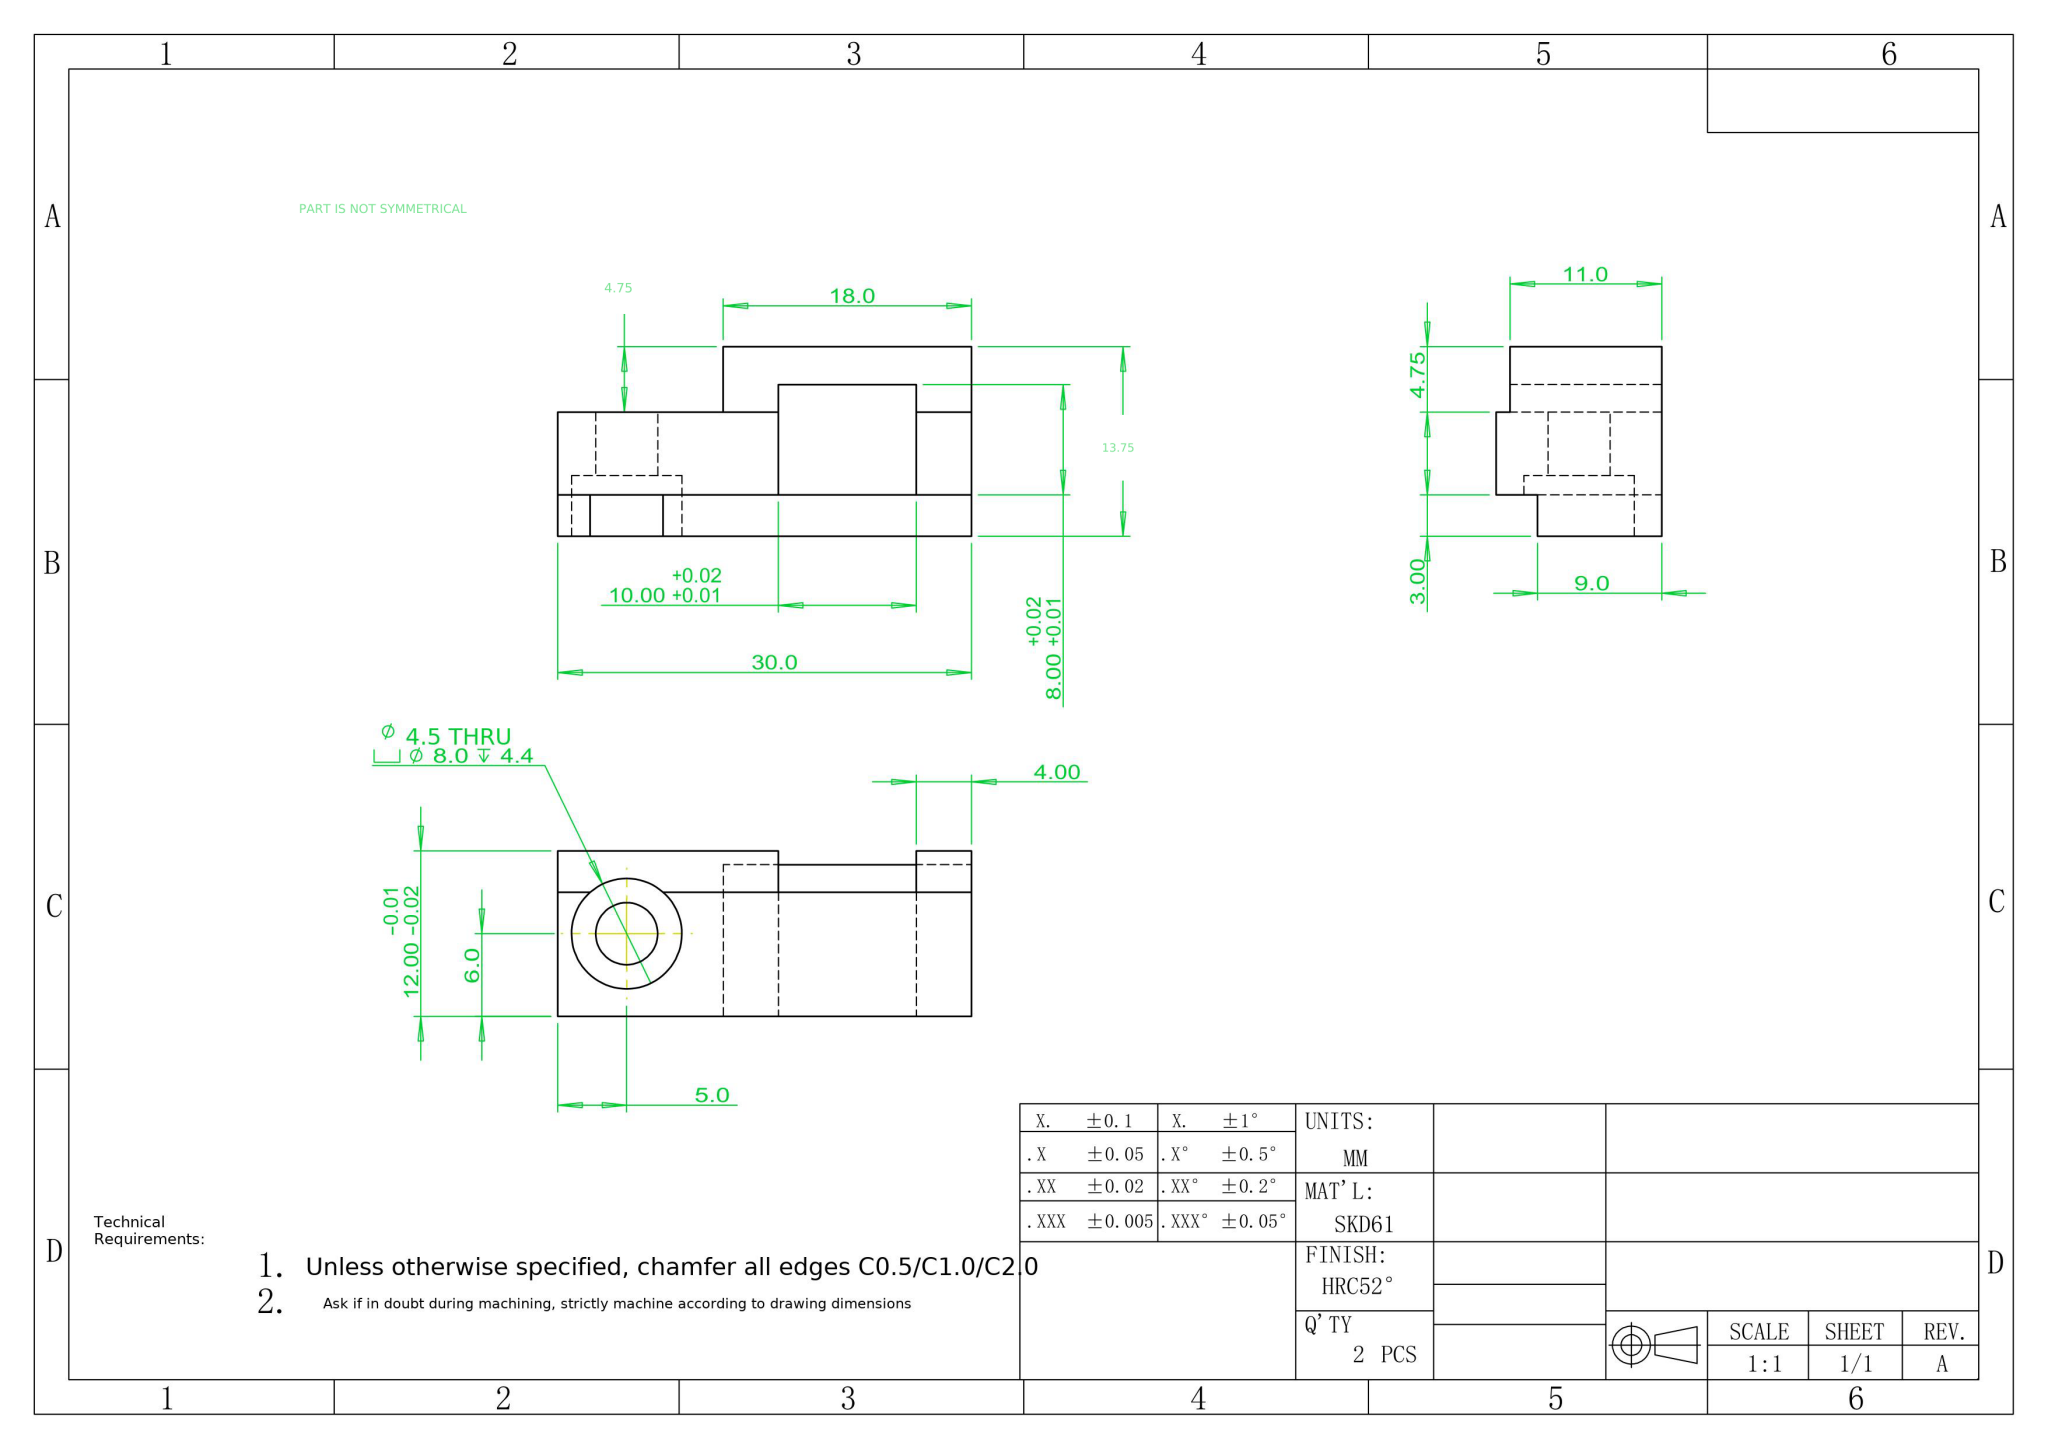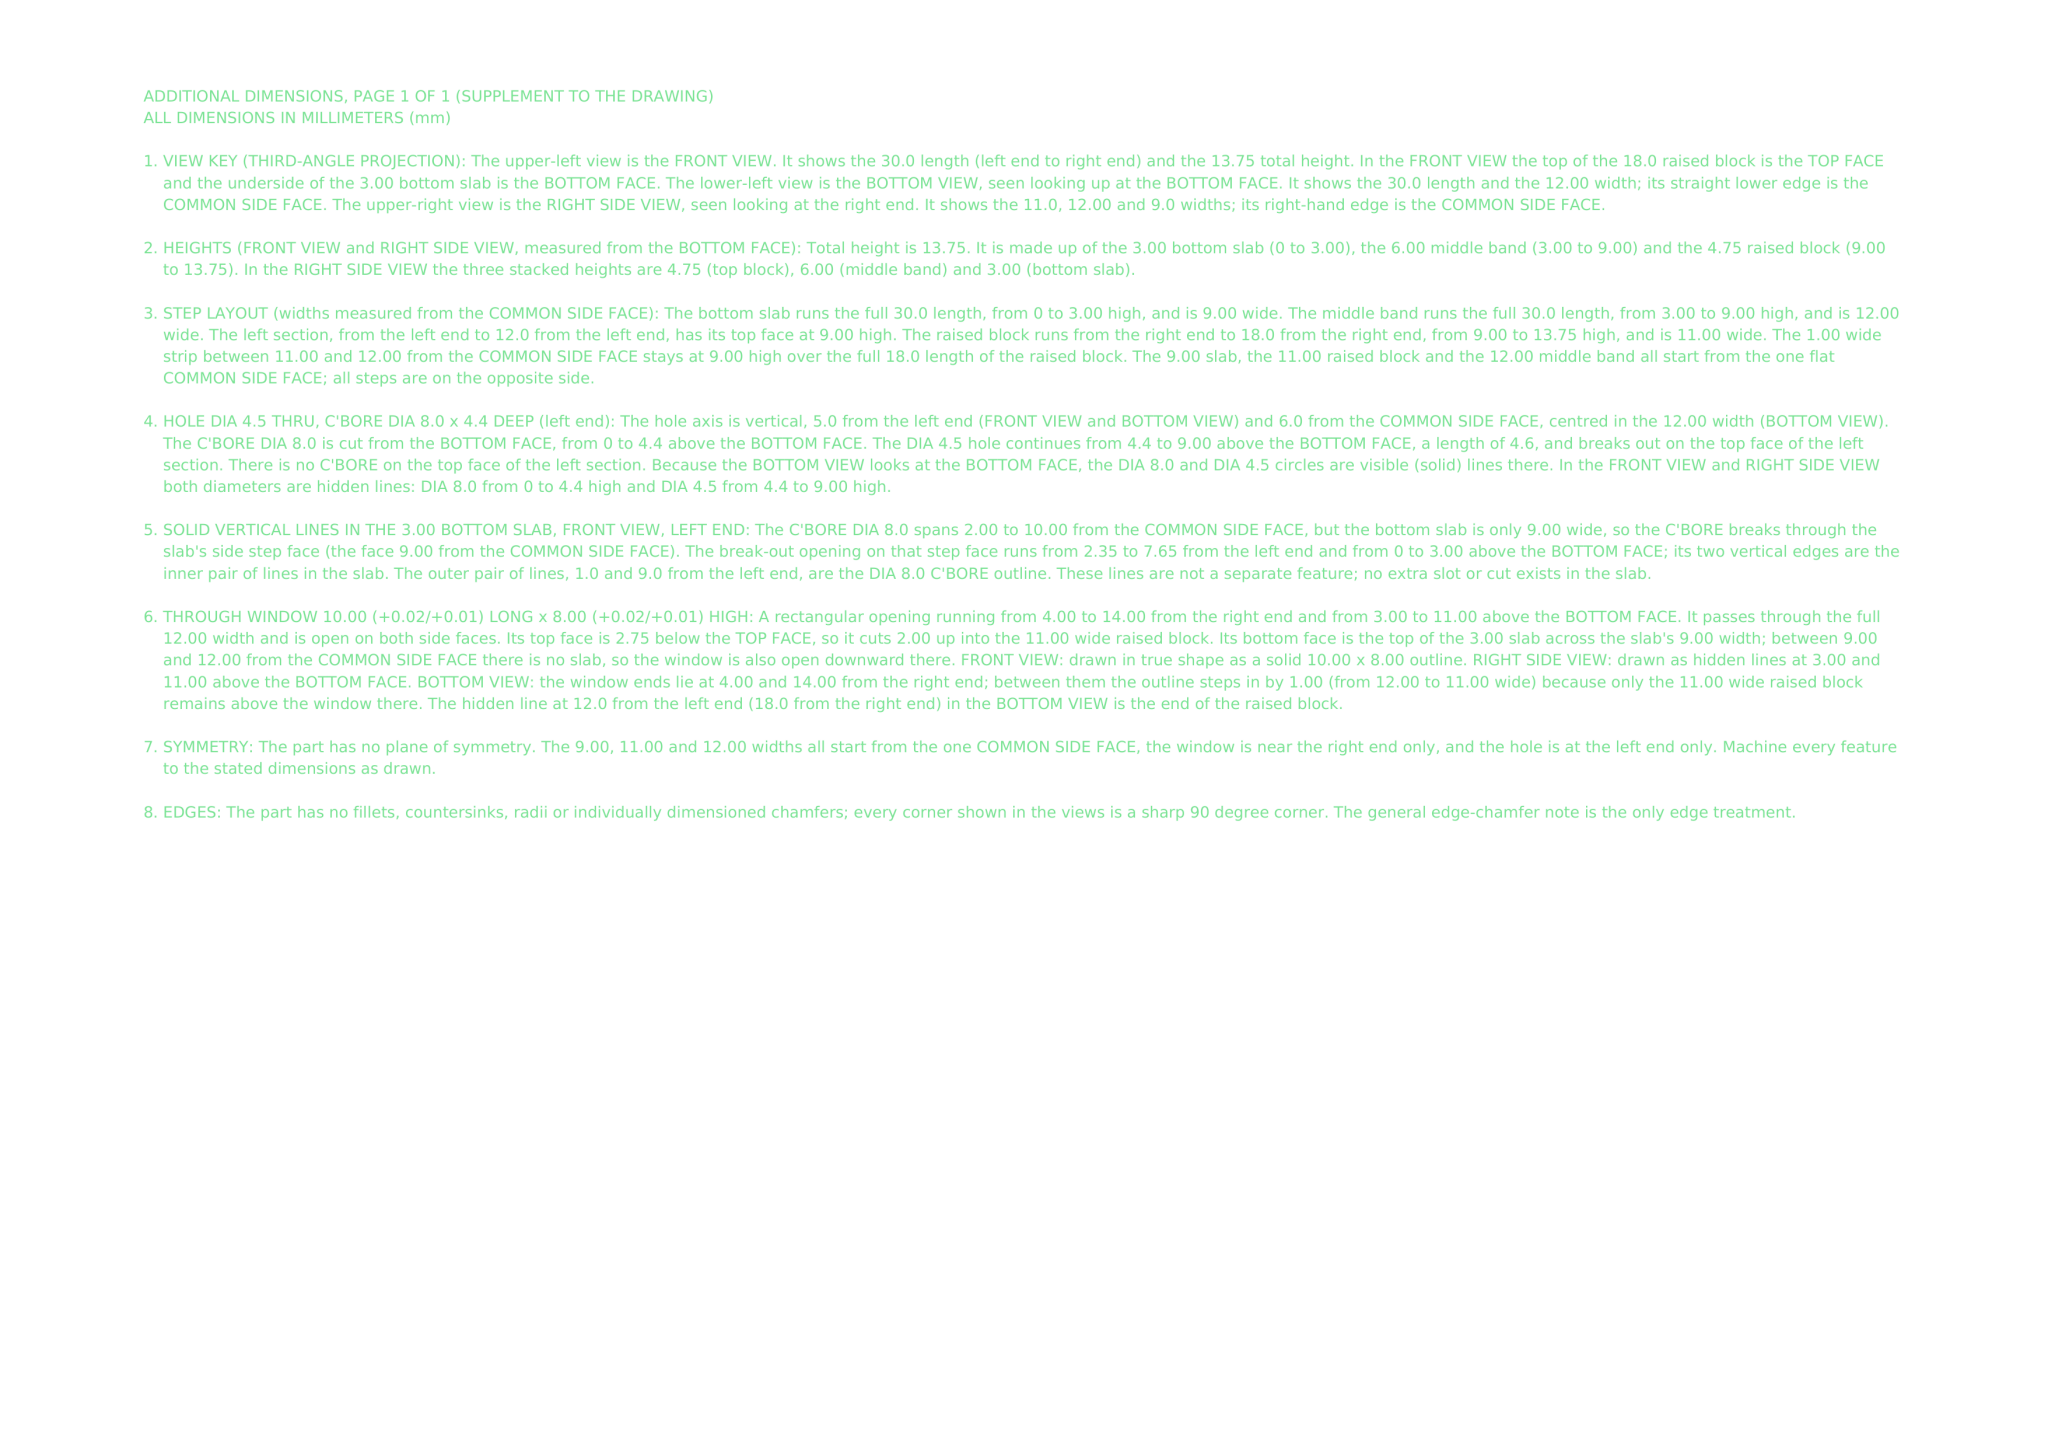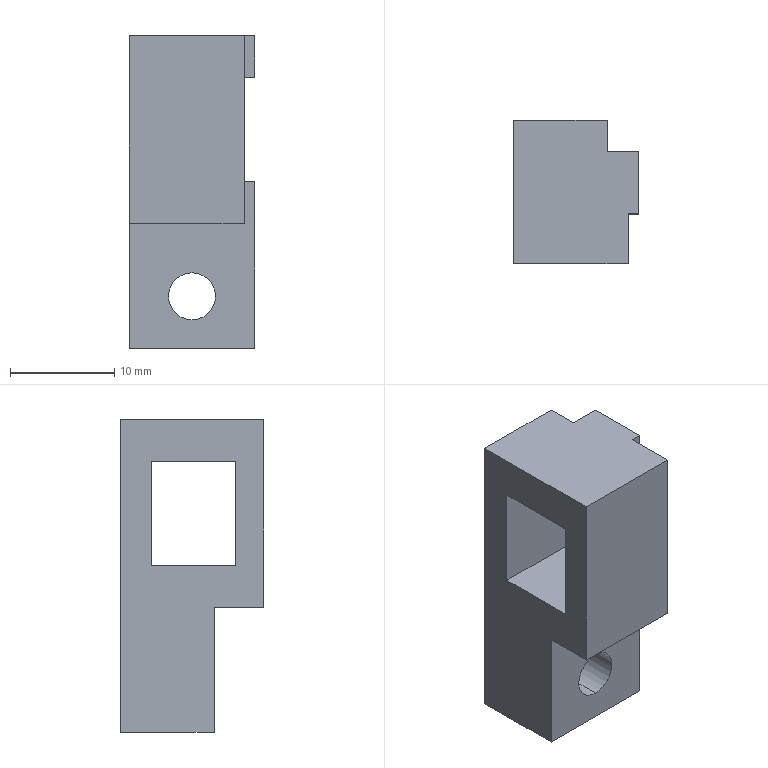Part | NX | mm | 1 solid | 24 faces | box 12 x 13.75 x 30 mm | volume 2687 mm3 | plane 20 | cylinder 4 | commonest cylinder face diameters 8 x2 4.5 x2
STEP:
#1=COLOUR_RGB('',0.9098,0.4431,0.03137);
#2=FILL_AREA_STYLE_COLOUR('',#1);
#3=FILL_AREA_STYLE('',(#2));
#4=SURFACE_STYLE_FILL_AREA(#3);
#5=SURFACE_SIDE_STYLE('',(#4));
#6=SURFACE_STYLE_USAGE(.BOTH.,#5);
#7=PRESENTATION_STYLE_ASSIGNMENT((#6));
#8=CARTESIAN_POINT('',(6.,4.6,-29.));
#9=VERTEX_POINT('',#8);
#10=CARTESIAN_POINT('',(6.,4.6,-21.));
#11=VERTEX_POINT('',#10);
#12=CARTESIAN_POINT('',(6.,4.6,-25.));
#13=DIRECTION('',(0.,1.,0.));
#14=DIRECTION('',(0.,0.,1.));
#15=AXIS2_PLACEMENT_3D('',#12,#13,#14);
#16=CIRCLE('',#15,4.);
#17=EDGE_CURVE('',#9,#11,#16,.T.);
#18=ORIENTED_EDGE('',*,*,#17,.F.);
#19=CARTESIAN_POINT('',(6.,9.,-29.));
#20=VERTEX_POINT('',#19);
#21=CARTESIAN_POINT('',(6.,9.,-29.));
#22=DIRECTION('',(0.,1.,0.));
#23=VECTOR('',#22,1000.);
#24=LINE('',#21,#23);
#25=EDGE_CURVE('',#9,#20,#24,.T.);
#26=ORIENTED_EDGE('',*,*,#25,.T.);
#27=CARTESIAN_POINT('',(6.,9.,-21.));
#28=VERTEX_POINT('',#27);
#29=CARTESIAN_POINT('',(6.,9.,-25.));
#30=DIRECTION('',(0.,1.,0.));
#31=DIRECTION('',(0.,0.,1.));
#32=AXIS2_PLACEMENT_3D('',#29,#30,#31);
#33=CIRCLE('',#32,4.);
#34=EDGE_CURVE('',#20,#28,#33,.T.);
#35=ORIENTED_EDGE('',*,*,#34,.T.);
#36=CARTESIAN_POINT('',(6.,9.,-21.));
#37=DIRECTION('',(0.,1.,0.));
#38=VECTOR('',#37,1000.);
#39=LINE('',#36,#38);
#40=EDGE_CURVE('',#11,#28,#39,.T.);
#41=ORIENTED_EDGE('',*,*,#40,.F.);
#42=EDGE_LOOP('',(#18,#26,#35,#41));
#43=FACE_OUTER_BOUND('',#42,.T.);
#44=CARTESIAN_POINT('',(6.,9.,-25.));
#45=DIRECTION('',(0.,1.,0.));
#46=DIRECTION('',(0.,0.,1.));
#47=AXIS2_PLACEMENT_3D('',#44,#45,#46);
#48=CYLINDRICAL_SURFACE('',#47,4.);
#49=ADVANCED_FACE('',(#43),#48,.F.);
#50=CARTESIAN_POINT('',(6.,0.,-27.25));
#51=VERTEX_POINT('',#50);
#52=CARTESIAN_POINT('',(6.,0.,-22.75));
#53=VERTEX_POINT('',#52);
#54=CARTESIAN_POINT('',(6.,0.,-25.));
#55=DIRECTION('',(0.,1.,0.));
#56=DIRECTION('',(0.,0.,1.));
#57=AXIS2_PLACEMENT_3D('',#54,#55,#56);
#58=CIRCLE('',#57,2.25);
#59=EDGE_CURVE('',#51,#53,#58,.T.);
#60=ORIENTED_EDGE('',*,*,#59,.F.);
#61=CARTESIAN_POINT('',(6.,4.6,-27.25));
#62=VERTEX_POINT('',#61);
#63=CARTESIAN_POINT('',(6.,9.,-27.25));
#64=DIRECTION('',(0.,1.,0.));
#65=VECTOR('',#64,1000.);
#66=LINE('',#63,#65);
#67=EDGE_CURVE('',#51,#62,#66,.T.);
#68=ORIENTED_EDGE('',*,*,#67,.T.);
#69=CARTESIAN_POINT('',(6.,4.6,-22.75));
#70=VERTEX_POINT('',#69);
#71=CARTESIAN_POINT('',(6.,4.6,-25.));
#72=DIRECTION('',(0.,1.,0.));
#73=DIRECTION('',(0.,0.,1.));
#74=AXIS2_PLACEMENT_3D('',#71,#72,#73);
#75=CIRCLE('',#74,2.25);
#76=EDGE_CURVE('',#62,#70,#75,.T.);
#77=ORIENTED_EDGE('',*,*,#76,.T.);
#78=CARTESIAN_POINT('',(6.,9.,-22.75));
#79=DIRECTION('',(0.,1.,0.));
#80=VECTOR('',#79,1000.);
#81=LINE('',#78,#80);
#82=EDGE_CURVE('',#53,#70,#81,.T.);
#83=ORIENTED_EDGE('',*,*,#82,.F.);
#84=EDGE_LOOP('',(#60,#68,#77,#83));
#85=FACE_OUTER_BOUND('',#84,.T.);
#86=CARTESIAN_POINT('',(6.,9.,-25.));
#87=DIRECTION('',(0.,1.,0.));
#88=DIRECTION('',(0.,0.,1.));
#89=AXIS2_PLACEMENT_3D('',#86,#87,#88);
#90=CYLINDRICAL_SURFACE('',#89,2.25);
#91=ADVANCED_FACE('',(#85),#90,.F.);
#92=CARTESIAN_POINT('',(12.,6.,0.));
#93=VERTEX_POINT('',#92);
#94=CARTESIAN_POINT('',(12.,-0.,0.));
#95=VERTEX_POINT('',#94);
#96=CARTESIAN_POINT('',(12.,0.,0.));
#97=DIRECTION('',(0.,-1.,0.));
#98=VECTOR('',#97,1000.);
#99=LINE('',#96,#98);
#100=EDGE_CURVE('',#93,#95,#99,.T.);
#101=ORIENTED_EDGE('',*,*,#100,.T.);
#102=CARTESIAN_POINT('',(12.,-0.,-4.));
#103=VERTEX_POINT('',#102);
#104=CARTESIAN_POINT('',(12.,-0.,0.));
#105=DIRECTION('',(0.,0.,1.));
#106=VECTOR('',#105,1000.);
#107=LINE('',#104,#106);
#108=EDGE_CURVE('',#103,#95,#107,.T.);
#109=ORIENTED_EDGE('',*,*,#108,.F.);
#110=CARTESIAN_POINT('',(12.,6.,-4.));
#111=VERTEX_POINT('',#110);
#112=CARTESIAN_POINT('',(12.,-2.,-4.));
#113=DIRECTION('',(0.,-1.,0.));
#114=VECTOR('',#113,1000.);
#115=LINE('',#112,#114);
#116=EDGE_CURVE('',#111,#103,#115,.T.);
#117=ORIENTED_EDGE('',*,*,#116,.F.);
#118=CARTESIAN_POINT('',(12.,6.,0.));
#119=DIRECTION('',(0.,0.,-1.));
#120=VECTOR('',#119,1000.);
#121=LINE('',#118,#120);
#122=EDGE_CURVE('',#93,#111,#121,.T.);
#123=ORIENTED_EDGE('',*,*,#122,.F.);
#124=EDGE_LOOP('',(#101,#109,#117,#123));
#125=FACE_OUTER_BOUND('',#124,.T.);
#126=CARTESIAN_POINT('',(12.,0.,0.));
#127=DIRECTION('',(-1.,0.,0.));
#128=DIRECTION('',(0.,0.,1.));
#129=AXIS2_PLACEMENT_3D('',#126,#127,#128);
#130=PLANE('',#129);
#131=ADVANCED_FACE('',(#125),#130,.F.);
#132=CARTESIAN_POINT('',(11.,-4.75,-18.));
#133=VERTEX_POINT('',#132);
#134=CARTESIAN_POINT('',(11.,-0.,-18.));
#135=VERTEX_POINT('',#134);
#136=CARTESIAN_POINT('',(11.,-0.,-18.));
#137=DIRECTION('',(0.,1.,0.));
#138=VECTOR('',#137,1000.);
#139=LINE('',#136,#138);
#140=EDGE_CURVE('',#133,#135,#139,.T.);
#141=ORIENTED_EDGE('',*,*,#140,.F.);
#142=CARTESIAN_POINT('',(0.,-4.75,-18.));
#143=VERTEX_POINT('',#142);
#144=CARTESIAN_POINT('',(0.,-4.75,-18.));
#145=DIRECTION('',(1.,0.,0.));
#146=VECTOR('',#145,1000.);
#147=LINE('',#144,#146);
#148=EDGE_CURVE('',#143,#133,#147,.T.);
#149=ORIENTED_EDGE('',*,*,#148,.F.);
#150=CARTESIAN_POINT('',(0.,0.,-18.));
#151=VERTEX_POINT('',#150);
#152=CARTESIAN_POINT('',(0.,-4.75,-18.));
#153=DIRECTION('',(0.,1.,0.));
#154=VECTOR('',#153,1000.);
#155=LINE('',#152,#154);
#156=EDGE_CURVE('',#143,#151,#155,.T.);
#157=ORIENTED_EDGE('',*,*,#156,.T.);
#158=CARTESIAN_POINT('',(0.,0.,-18.));
#159=DIRECTION('',(1.,0.,0.));
#160=VECTOR('',#159,1000.);
#161=LINE('',#158,#160);
#162=EDGE_CURVE('',#151,#135,#161,.T.);
#163=ORIENTED_EDGE('',*,*,#162,.T.);
#164=EDGE_LOOP('',(#141,#149,#157,#163));
#165=FACE_OUTER_BOUND('',#164,.T.);
#166=CARTESIAN_POINT('',(0.,-4.75,-18.));
#167=DIRECTION('',(0.,0.,1.));
#168=DIRECTION('',(1.,0.,0.));
#169=AXIS2_PLACEMENT_3D('',#166,#167,#168);
#170=PLANE('',#169);
#171=ADVANCED_FACE('',(#165),#170,.F.);
#172=ORIENTED_EDGE('',*,*,#148,.T.);
#173=CARTESIAN_POINT('',(11.,-4.75,0.));
#174=VERTEX_POINT('',#173);
#175=CARTESIAN_POINT('',(11.,-4.75,0.));
#176=DIRECTION('',(0.,0.,-1.));
#177=VECTOR('',#176,1000.);
#178=LINE('',#175,#177);
#179=EDGE_CURVE('',#174,#133,#178,.T.);
#180=ORIENTED_EDGE('',*,*,#179,.F.);
#181=CARTESIAN_POINT('',(0.,-4.75,0.));
#182=VERTEX_POINT('',#181);
#183=CARTESIAN_POINT('',(0.,-4.75,0.));
#184=DIRECTION('',(-1.,0.,0.));
#185=VECTOR('',#184,1000.);
#186=LINE('',#183,#185);
#187=EDGE_CURVE('',#174,#182,#186,.T.);
#188=ORIENTED_EDGE('',*,*,#187,.T.);
#189=CARTESIAN_POINT('',(0.,-4.75,0.));
#190=DIRECTION('',(0.,0.,-1.));
#191=VECTOR('',#190,1000.);
#192=LINE('',#189,#191);
#193=EDGE_CURVE('',#182,#143,#192,.T.);
#194=ORIENTED_EDGE('',*,*,#193,.T.);
#195=EDGE_LOOP('',(#172,#180,#188,#194));
#196=FACE_OUTER_BOUND('',#195,.T.);
#197=CARTESIAN_POINT('',(0.,-4.75,0.));
#198=DIRECTION('',(0.,-1.,0.));
#199=DIRECTION('',(0.,0.,-1.));
#200=AXIS2_PLACEMENT_3D('',#197,#198,#199);
#201=PLANE('',#200);
#202=ADVANCED_FACE('',(#196),#201,.T.);
#203=CARTESIAN_POINT('',(11.,-2.,-14.));
#204=VERTEX_POINT('',#203);
#205=CARTESIAN_POINT('',(11.,-2.,-4.));
#206=VERTEX_POINT('',#205);
#207=CARTESIAN_POINT('',(11.,-2.,-14.));
#208=DIRECTION('',(0.,-0.,1.));
#209=VECTOR('',#208,1000.);
#210=LINE('',#207,#209);
#211=EDGE_CURVE('',#204,#206,#210,.T.);
#212=ORIENTED_EDGE('',*,*,#211,.F.);
#213=CARTESIAN_POINT('',(0.,-2.,-14.));
#214=VERTEX_POINT('',#213);
#215=CARTESIAN_POINT('',(-18.,-2.,-14.));
#216=DIRECTION('',(1.,0.,0.));
#217=VECTOR('',#216,1000.);
#218=LINE('',#215,#217);
#219=EDGE_CURVE('',#214,#204,#218,.T.);
#220=ORIENTED_EDGE('',*,*,#219,.F.);
#221=CARTESIAN_POINT('',(0.,-2.,-4.));
#222=VERTEX_POINT('',#221);
#223=CARTESIAN_POINT('',(0.,-2.,-0.));
#224=DIRECTION('',(0.,-0.,1.));
#225=VECTOR('',#224,1000.);
#226=LINE('',#223,#225);
#227=EDGE_CURVE('',#214,#222,#226,.T.);
#228=ORIENTED_EDGE('',*,*,#227,.T.);
#229=CARTESIAN_POINT('',(-18.,-2.,-4.));
#230=DIRECTION('',(1.,0.,0.));
#231=VECTOR('',#230,1000.);
#232=LINE('',#229,#231);
#233=EDGE_CURVE('',#222,#206,#232,.T.);
#234=ORIENTED_EDGE('',*,*,#233,.T.);
#235=EDGE_LOOP('',(#212,#220,#228,#234));
#236=FACE_OUTER_BOUND('',#235,.T.);
#237=CARTESIAN_POINT('',(-18.,-2.,-14.));
#238=DIRECTION('',(0.,-1.,-0.));
#239=DIRECTION('',(0.,0.,-1.));
#240=AXIS2_PLACEMENT_3D('',#237,#238,#239);
#241=PLANE('',#240);
#242=ADVANCED_FACE('',(#236),#241,.F.);
#243=CARTESIAN_POINT('',(12.,-0.,-14.));
#244=VERTEX_POINT('',#243);
#245=CARTESIAN_POINT('',(12.,6.,-14.));
#246=VERTEX_POINT('',#245);
#247=CARTESIAN_POINT('',(12.,-2.,-14.));
#248=DIRECTION('',(0.,1.,0.));
#249=VECTOR('',#248,1000.);
#250=LINE('',#247,#249);
#251=EDGE_CURVE('',#244,#246,#250,.T.);
#252=ORIENTED_EDGE('',*,*,#251,.F.);
#253=CARTESIAN_POINT('',(12.,0.,-30.));
#254=VERTEX_POINT('',#253);
#255=CARTESIAN_POINT('',(12.,0.,0.));
#256=DIRECTION('',(0.,0.,-1.));
#257=VECTOR('',#256,1000.);
#258=LINE('',#255,#257);
#259=EDGE_CURVE('',#244,#254,#258,.T.);
#260=ORIENTED_EDGE('',*,*,#259,.T.);
#261=CARTESIAN_POINT('',(12.,6.,-30.));
#262=VERTEX_POINT('',#261);
#263=CARTESIAN_POINT('',(12.,0.,-30.));
#264=DIRECTION('',(0.,1.,0.));
#265=VECTOR('',#264,1000.);
#266=LINE('',#263,#265);
#267=EDGE_CURVE('',#254,#262,#266,.T.);
#268=ORIENTED_EDGE('',*,*,#267,.T.);
#269=CARTESIAN_POINT('',(12.,6.,0.));
#270=DIRECTION('',(0.,0.,-1.));
#271=VECTOR('',#270,1000.);
#272=LINE('',#269,#271);
#273=EDGE_CURVE('',#246,#262,#272,.T.);
#274=ORIENTED_EDGE('',*,*,#273,.F.);
#275=EDGE_LOOP('',(#252,#260,#268,#274));
#276=FACE_OUTER_BOUND('',#275,.T.);
#277=CARTESIAN_POINT('',(12.,0.,0.));
#278=DIRECTION('',(-1.,0.,0.));
#279=DIRECTION('',(0.,0.,1.));
#280=AXIS2_PLACEMENT_3D('',#277,#278,#279);
#281=PLANE('',#280);
#282=ADVANCED_FACE('',(#276),#281,.F.);
#283=CARTESIAN_POINT('',(6.,0.,-25.));
#284=DIRECTION('',(0.,1.,0.));
#285=DIRECTION('',(0.,0.,1.));
#286=AXIS2_PLACEMENT_3D('',#283,#284,#285);
#287=CIRCLE('',#286,2.25);
#288=EDGE_CURVE('',#53,#51,#287,.T.);
#289=ORIENTED_EDGE('',*,*,#288,.T.);
#290=ORIENTED_EDGE('',*,*,#59,.T.);
#291=EDGE_LOOP('',(#289,#290));
#292=FACE_BOUND('',#291,.T.);
#293=ORIENTED_EDGE('',*,*,#162,.F.);
#294=CARTESIAN_POINT('',(0.,0.,-30.));
#295=VERTEX_POINT('',#294);
#296=CARTESIAN_POINT('',(0.,0.,0.));
#297=DIRECTION('',(0.,0.,-1.));
#298=VECTOR('',#297,1000.);
#299=LINE('',#296,#298);
#300=EDGE_CURVE('',#151,#295,#299,.T.);
#301=ORIENTED_EDGE('',*,*,#300,.T.);
#302=CARTESIAN_POINT('',(12.,0.,-30.));
#303=DIRECTION('',(-1.,0.,0.));
#304=VECTOR('',#303,1000.);
#305=LINE('',#302,#304);
#306=EDGE_CURVE('',#254,#295,#305,.T.);
#307=ORIENTED_EDGE('',*,*,#306,.F.);
#308=ORIENTED_EDGE('',*,*,#259,.F.);
#309=CARTESIAN_POINT('',(11.,-0.,-14.));
#310=VERTEX_POINT('',#309);
#311=CARTESIAN_POINT('',(-18.,-0.,-14.));
#312=DIRECTION('',(1.,0.,0.));
#313=VECTOR('',#312,1000.);
#314=LINE('',#311,#313);
#315=EDGE_CURVE('',#310,#244,#314,.T.);
#316=ORIENTED_EDGE('',*,*,#315,.F.);
#317=CARTESIAN_POINT('',(11.,-0.,0.));
#318=DIRECTION('',(0.,0.,1.));
#319=VECTOR('',#318,1000.);
#320=LINE('',#317,#319);
#321=EDGE_CURVE('',#135,#310,#320,.T.);
#322=ORIENTED_EDGE('',*,*,#321,.F.);
#323=EDGE_LOOP('',(#293,#301,#307,#308,#316,#322));
#324=FACE_OUTER_BOUND('',#323,.T.);
#325=CARTESIAN_POINT('',(12.,0.,0.));
#326=DIRECTION('',(0.,1.,0.));
#327=DIRECTION('',(0.,0.,1.));
#328=AXIS2_PLACEMENT_3D('',#325,#326,#327);
#329=PLANE('',#328);
#330=ADVANCED_FACE('',(#292,#324),#329,.F.);
#331=CARTESIAN_POINT('',(11.,-0.,0.));
#332=VERTEX_POINT('',#331);
#333=CARTESIAN_POINT('',(11.,-0.,0.));
#334=DIRECTION('',(0.,-1.,0.));
#335=VECTOR('',#334,1000.);
#336=LINE('',#333,#335);
#337=EDGE_CURVE('',#332,#174,#336,.T.);
#338=ORIENTED_EDGE('',*,*,#337,.F.);
#339=CARTESIAN_POINT('',(11.,-0.,0.));
#340=DIRECTION('',(1.,0.,0.));
#341=VECTOR('',#340,1000.);
#342=LINE('',#339,#341);
#343=EDGE_CURVE('',#332,#95,#342,.T.);
#344=ORIENTED_EDGE('',*,*,#343,.T.);
#345=ORIENTED_EDGE('',*,*,#100,.F.);
#346=CARTESIAN_POINT('',(9.,6.,0.));
#347=VERTEX_POINT('',#346);
#348=CARTESIAN_POINT('',(12.,6.,0.));
#349=DIRECTION('',(1.,0.,-0.));
#350=VECTOR('',#349,1000.);
#351=LINE('',#348,#350);
#352=EDGE_CURVE('',#347,#93,#351,.T.);
#353=ORIENTED_EDGE('',*,*,#352,.F.);
#354=CARTESIAN_POINT('',(9.,9.,0.));
#355=VERTEX_POINT('',#354);
#356=CARTESIAN_POINT('',(9.,6.,0.));
#357=DIRECTION('',(0.,1.,0.));
#358=VECTOR('',#357,1000.);
#359=LINE('',#356,#358);
#360=EDGE_CURVE('',#347,#355,#359,.T.);
#361=ORIENTED_EDGE('',*,*,#360,.T.);
#362=CARTESIAN_POINT('',(0.,9.,0.));
#363=VERTEX_POINT('',#362);
#364=CARTESIAN_POINT('',(12.,9.,0.));
#365=DIRECTION('',(-1.,0.,0.));
#366=VECTOR('',#365,1000.);
#367=LINE('',#364,#366);
#368=EDGE_CURVE('',#355,#363,#367,.T.);
#369=ORIENTED_EDGE('',*,*,#368,.T.);
#370=CARTESIAN_POINT('',(0.,0.,0.));
#371=DIRECTION('',(0.,-1.,0.));
#372=VECTOR('',#371,1000.);
#373=LINE('',#370,#372);
#374=EDGE_CURVE('',#363,#182,#373,.T.);
#375=ORIENTED_EDGE('',*,*,#374,.T.);
#376=ORIENTED_EDGE('',*,*,#187,.F.);
#377=EDGE_LOOP('',(#338,#344,#345,#353,#361,#369,#375,#376));
#378=FACE_OUTER_BOUND('',#377,.T.);
#379=CARTESIAN_POINT('',(12.,0.,0.));
#380=DIRECTION('',(0.,0.,-1.));
#381=DIRECTION('',(-1.,0.,0.));
#382=AXIS2_PLACEMENT_3D('',#379,#380,#381);
#383=PLANE('',#382);
#384=ADVANCED_FACE('',(#378),#383,.F.);
#385=CARTESIAN_POINT('',(9.,9.,-30.));
#386=VERTEX_POINT('',#385);
#387=CARTESIAN_POINT('',(0.,9.,-30.));
#388=VERTEX_POINT('',#387);
#389=CARTESIAN_POINT('',(12.,9.,-30.));
#390=DIRECTION('',(-1.,0.,0.));
#391=VECTOR('',#390,1000.);
#392=LINE('',#389,#391);
#393=EDGE_CURVE('',#386,#388,#392,.T.);
#394=ORIENTED_EDGE('',*,*,#393,.F.);
#395=CARTESIAN_POINT('',(9.,6.,-30.));
#396=VERTEX_POINT('',#395);
#397=CARTESIAN_POINT('',(9.,6.,-30.));
#398=DIRECTION('',(0.,1.,0.));
#399=VECTOR('',#398,1000.);
#400=LINE('',#397,#399);
#401=EDGE_CURVE('',#396,#386,#400,.T.);
#402=ORIENTED_EDGE('',*,*,#401,.F.);
#403=CARTESIAN_POINT('',(12.,6.,-30.));
#404=DIRECTION('',(-1.,0.,0.));
#405=VECTOR('',#404,1000.);
#406=LINE('',#403,#405);
#407=EDGE_CURVE('',#262,#396,#406,.T.);
#408=ORIENTED_EDGE('',*,*,#407,.F.);
#409=ORIENTED_EDGE('',*,*,#267,.F.);
#410=ORIENTED_EDGE('',*,*,#306,.T.);
#411=CARTESIAN_POINT('',(0.,0.,-30.));
#412=DIRECTION('',(0.,1.,0.));
#413=VECTOR('',#412,1000.);
#414=LINE('',#411,#413);
#415=EDGE_CURVE('',#295,#388,#414,.T.);
#416=ORIENTED_EDGE('',*,*,#415,.T.);
#417=EDGE_LOOP('',(#394,#402,#408,#409,#410,#416));
#418=FACE_OUTER_BOUND('',#417,.T.);
#419=CARTESIAN_POINT('',(12.,0.,-30.));
#420=DIRECTION('',(0.,0.,1.));
#421=DIRECTION('',(1.,0.,0.));
#422=AXIS2_PLACEMENT_3D('',#419,#420,#421);
#423=PLANE('',#422);
#424=ADVANCED_FACE('',(#418),#423,.F.);
#425=ORIENTED_EDGE('',*,*,#368,.F.);
#426=CARTESIAN_POINT('',(9.,9.,-22.354));
#427=VERTEX_POINT('',#426);
#428=CARTESIAN_POINT('',(9.,9.,0.));
#429=DIRECTION('',(0.,0.,1.));
#430=VECTOR('',#429,1000.);
#431=LINE('',#428,#430);
#432=EDGE_CURVE('',#427,#355,#431,.T.);
#433=ORIENTED_EDGE('',*,*,#432,.F.);
#434=CARTESIAN_POINT('',(6.,9.,-25.));
#435=DIRECTION('',(0.,1.,0.));
#436=DIRECTION('',(0.,0.,1.));
#437=AXIS2_PLACEMENT_3D('',#434,#435,#436);
#438=CIRCLE('',#437,4.);
#439=EDGE_CURVE('',#28,#427,#438,.T.);
#440=ORIENTED_EDGE('',*,*,#439,.F.);
#441=ORIENTED_EDGE('',*,*,#34,.F.);
#442=CARTESIAN_POINT('',(9.,9.,-27.646));
#443=VERTEX_POINT('',#442);
#444=CARTESIAN_POINT('',(6.,9.,-25.));
#445=DIRECTION('',(0.,1.,0.));
#446=DIRECTION('',(0.,0.,1.));
#447=AXIS2_PLACEMENT_3D('',#444,#445,#446);
#448=CIRCLE('',#447,4.);
#449=EDGE_CURVE('',#443,#20,#448,.T.);
#450=ORIENTED_EDGE('',*,*,#449,.F.);
#451=CARTESIAN_POINT('',(9.,9.,0.));
#452=DIRECTION('',(0.,0.,1.));
#453=VECTOR('',#452,1000.);
#454=LINE('',#451,#453);
#455=EDGE_CURVE('',#386,#443,#454,.T.);
#456=ORIENTED_EDGE('',*,*,#455,.F.);
#457=ORIENTED_EDGE('',*,*,#393,.T.);
#458=CARTESIAN_POINT('',(0.,9.,0.));
#459=DIRECTION('',(0.,0.,1.));
#460=VECTOR('',#459,1000.);
#461=LINE('',#458,#460);
#462=EDGE_CURVE('',#388,#363,#461,.T.);
#463=ORIENTED_EDGE('',*,*,#462,.T.);
#464=EDGE_LOOP('',(#425,#433,#440,#441,#450,#456,#457,#463));
#465=FACE_OUTER_BOUND('',#464,.T.);
#466=CARTESIAN_POINT('',(12.,9.,0.));
#467=DIRECTION('',(0.,-1.,0.));
#468=DIRECTION('',(0.,0.,-1.));
#469=AXIS2_PLACEMENT_3D('',#466,#467,#468);
#470=PLANE('',#469);
#471=ADVANCED_FACE('',(#465),#470,.F.);
#472=CARTESIAN_POINT('',(0.,6.,-14.));
#473=VERTEX_POINT('',#472);
#474=CARTESIAN_POINT('',(0.,0.,-14.));
#475=DIRECTION('',(0.,-1.,-0.));
#476=VECTOR('',#475,1000.);
#477=LINE('',#474,#476);
#478=EDGE_CURVE('',#473,#214,#477,.T.);
#479=ORIENTED_EDGE('',*,*,#478,.F.);
#480=CARTESIAN_POINT('',(0.,6.,-4.));
#481=VERTEX_POINT('',#480);
#482=CARTESIAN_POINT('',(0.,6.,0.));
#483=DIRECTION('',(0.,0.,-1.));
#484=VECTOR('',#483,1000.);
#485=LINE('',#482,#484);
#486=EDGE_CURVE('',#481,#473,#485,.T.);
#487=ORIENTED_EDGE('',*,*,#486,.F.);
#488=CARTESIAN_POINT('',(0.,0.,-4.));
#489=DIRECTION('',(0.,1.,0.));
#490=VECTOR('',#489,1000.);
#491=LINE('',#488,#490);
#492=EDGE_CURVE('',#222,#481,#491,.T.);
#493=ORIENTED_EDGE('',*,*,#492,.F.);
#494=ORIENTED_EDGE('',*,*,#227,.F.);
#495=EDGE_LOOP('',(#479,#487,#493,#494));
#496=FACE_BOUND('',#495,.T.);
#497=ORIENTED_EDGE('',*,*,#374,.F.);
#498=ORIENTED_EDGE('',*,*,#462,.F.);
#499=ORIENTED_EDGE('',*,*,#415,.F.);
#500=ORIENTED_EDGE('',*,*,#300,.F.);
#501=ORIENTED_EDGE('',*,*,#156,.F.);
#502=ORIENTED_EDGE('',*,*,#193,.F.);
#503=EDGE_LOOP('',(#497,#498,#499,#500,#501,#502));
#504=FACE_OUTER_BOUND('',#503,.T.);
#505=CARTESIAN_POINT('',(0.,0.,0.));
#506=DIRECTION('',(-1.,0.,0.));
#507=DIRECTION('',(0.,0.,1.));
#508=AXIS2_PLACEMENT_3D('',#505,#506,#507);
#509=PLANE('',#508);
#510=ADVANCED_FACE('',(#496,#504),#509,.T.);
#511=CARTESIAN_POINT('',(11.,-2.,-14.));
#512=DIRECTION('',(0.,-1.,-0.));
#513=VECTOR('',#512,1000.);
#514=LINE('',#511,#513);
#515=EDGE_CURVE('',#310,#204,#514,.T.);
#516=ORIENTED_EDGE('',*,*,#515,.F.);
#517=ORIENTED_EDGE('',*,*,#315,.T.);
#518=ORIENTED_EDGE('',*,*,#251,.T.);
#519=CARTESIAN_POINT('',(9.,6.,-14.));
#520=VERTEX_POINT('',#519);
#521=CARTESIAN_POINT('',(-18.,6.,-14.));
#522=DIRECTION('',(1.,0.,0.));
#523=VECTOR('',#522,1000.);
#524=LINE('',#521,#523);
#525=EDGE_CURVE('',#520,#246,#524,.T.);
#526=ORIENTED_EDGE('',*,*,#525,.F.);
#527=CARTESIAN_POINT('',(-18.,6.,-14.));
#528=DIRECTION('',(1.,0.,0.));
#529=VECTOR('',#528,1000.);
#530=LINE('',#527,#529);
#531=EDGE_CURVE('',#473,#520,#530,.T.);
#532=ORIENTED_EDGE('',*,*,#531,.F.);
#533=ORIENTED_EDGE('',*,*,#478,.T.);
#534=ORIENTED_EDGE('',*,*,#219,.T.);
#535=EDGE_LOOP('',(#516,#517,#518,#526,#532,#533,#534));
#536=FACE_OUTER_BOUND('',#535,.T.);
#537=CARTESIAN_POINT('',(-18.,-2.,-14.));
#538=DIRECTION('',(0.,0.,-1.));
#539=DIRECTION('',(0.,1.,0.));
#540=AXIS2_PLACEMENT_3D('',#537,#538,#539);
#541=PLANE('',#540);
#542=ADVANCED_FACE('',(#536),#541,.F.);
#543=ORIENTED_EDGE('',*,*,#116,.T.);
#544=CARTESIAN_POINT('',(11.,-0.,-4.));
#545=VERTEX_POINT('',#544);
#546=CARTESIAN_POINT('',(-18.,-0.,-4.));
#547=DIRECTION('',(-1.,0.,0.));
#548=VECTOR('',#547,1000.);
#549=LINE('',#546,#548);
#550=EDGE_CURVE('',#103,#545,#549,.T.);
#551=ORIENTED_EDGE('',*,*,#550,.T.);
#552=CARTESIAN_POINT('',(11.,-2.,-4.));
#553=DIRECTION('',(0.,1.,0.));
#554=VECTOR('',#553,1000.);
#555=LINE('',#552,#554);
#556=EDGE_CURVE('',#206,#545,#555,.T.);
#557=ORIENTED_EDGE('',*,*,#556,.F.);
#558=ORIENTED_EDGE('',*,*,#233,.F.);
#559=ORIENTED_EDGE('',*,*,#492,.T.);
#560=CARTESIAN_POINT('',(9.,6.,-4.));
#561=VERTEX_POINT('',#560);
#562=CARTESIAN_POINT('',(-18.,6.,-4.));
#563=DIRECTION('',(1.,0.,0.));
#564=VECTOR('',#563,1000.);
#565=LINE('',#562,#564);
#566=EDGE_CURVE('',#481,#561,#565,.T.);
#567=ORIENTED_EDGE('',*,*,#566,.T.);
#568=CARTESIAN_POINT('',(-18.,6.,-4.));
#569=DIRECTION('',(-1.,0.,0.));
#570=VECTOR('',#569,1000.);
#571=LINE('',#568,#570);
#572=EDGE_CURVE('',#111,#561,#571,.T.);
#573=ORIENTED_EDGE('',*,*,#572,.F.);
#574=EDGE_LOOP('',(#543,#551,#557,#558,#559,#567,#573));
#575=FACE_OUTER_BOUND('',#574,.T.);
#576=CARTESIAN_POINT('',(-18.,-2.,-4.));
#577=DIRECTION('',(0.,0.,1.));
#578=DIRECTION('',(1.,0.,0.));
#579=AXIS2_PLACEMENT_3D('',#576,#577,#578);
#580=PLANE('',#579);
#581=ADVANCED_FACE('',(#575),#580,.F.);
#582=ORIENTED_EDGE('',*,*,#531,.T.);
#583=CARTESIAN_POINT('',(9.,6.,0.));
#584=DIRECTION('',(0.,0.,1.));
#585=VECTOR('',#584,1000.);
#586=LINE('',#583,#585);
#587=EDGE_CURVE('',#520,#561,#586,.T.);
#588=ORIENTED_EDGE('',*,*,#587,.T.);
#589=ORIENTED_EDGE('',*,*,#566,.F.);
#590=ORIENTED_EDGE('',*,*,#486,.T.);
#591=EDGE_LOOP('',(#582,#588,#589,#590));
#592=FACE_OUTER_BOUND('',#591,.T.);
#593=CARTESIAN_POINT('',(-18.,6.,-14.));
#594=DIRECTION('',(0.,1.,0.));
#595=DIRECTION('',(0.,0.,1.));
#596=AXIS2_PLACEMENT_3D('',#593,#594,#595);
#597=PLANE('',#596);
#598=ADVANCED_FACE('',(#592),#597,.F.);
#599=ORIENTED_EDGE('',*,*,#67,.F.);
#600=ORIENTED_EDGE('',*,*,#288,.F.);
#601=ORIENTED_EDGE('',*,*,#82,.T.);
#602=CARTESIAN_POINT('',(6.,4.6,-25.));
#603=DIRECTION('',(0.,1.,0.));
#604=DIRECTION('',(0.,0.,1.));
#605=AXIS2_PLACEMENT_3D('',#602,#603,#604);
#606=CIRCLE('',#605,2.25);
#607=EDGE_CURVE('',#70,#62,#606,.T.);
#608=ORIENTED_EDGE('',*,*,#607,.T.);
#609=EDGE_LOOP('',(#599,#600,#601,#608));
#610=FACE_OUTER_BOUND('',#609,.T.);
#611=CARTESIAN_POINT('',(6.,9.,-25.));
#612=DIRECTION('',(0.,1.,0.));
#613=DIRECTION('',(0.,0.,1.));
#614=AXIS2_PLACEMENT_3D('',#611,#612,#613);
#615=CYLINDRICAL_SURFACE('',#614,2.25);
#616=ADVANCED_FACE('',(#610),#615,.F.);
#617=ORIENTED_EDGE('',*,*,#607,.F.);
#618=ORIENTED_EDGE('',*,*,#76,.F.);
#619=EDGE_LOOP('',(#617,#618));
#620=FACE_BOUND('',#619,.T.);
#621=CARTESIAN_POINT('',(6.,4.6,-25.));
#622=DIRECTION('',(0.,1.,0.));
#623=DIRECTION('',(0.,0.,1.));
#624=AXIS2_PLACEMENT_3D('',#621,#622,#623);
#625=CIRCLE('',#624,4.);
#626=EDGE_CURVE('',#11,#9,#625,.T.);
#627=ORIENTED_EDGE('',*,*,#626,.T.);
#628=ORIENTED_EDGE('',*,*,#17,.T.);
#629=EDGE_LOOP('',(#627,#628));
#630=FACE_OUTER_BOUND('',#629,.T.);
#631=CARTESIAN_POINT('',(8.25,4.6,-25.));
#632=DIRECTION('',(0.,-1.,0.));
#633=DIRECTION('',(0.,0.,-1.));
#634=AXIS2_PLACEMENT_3D('',#631,#632,#633);
#635=PLANE('',#634);
#636=ADVANCED_FACE('',(#620,#630),#635,.F.);
#637=ORIENTED_EDGE('',*,*,#25,.F.);
#638=ORIENTED_EDGE('',*,*,#626,.F.);
#639=ORIENTED_EDGE('',*,*,#40,.T.);
#640=ORIENTED_EDGE('',*,*,#439,.T.);
#641=CARTESIAN_POINT('',(9.,6.,-22.354));
#642=VERTEX_POINT('',#641);
#643=CARTESIAN_POINT('',(9.,9.,-22.354));
#644=DIRECTION('',(0.,-1.,0.));
#645=VECTOR('',#644,1000.);
#646=LINE('',#643,#645);
#647=EDGE_CURVE('',#427,#642,#646,.T.);
#648=ORIENTED_EDGE('',*,*,#647,.T.);
#649=CARTESIAN_POINT('',(9.,6.,-27.646));
#650=VERTEX_POINT('',#649);
#651=CARTESIAN_POINT('',(6.,6.,-25.));
#652=DIRECTION('',(0.,-1.,0.));
#653=DIRECTION('',(0.,0.,1.));
#654=AXIS2_PLACEMENT_3D('',#651,#652,#653);
#655=CIRCLE('',#654,4.);
#656=EDGE_CURVE('',#650,#642,#655,.T.);
#657=ORIENTED_EDGE('',*,*,#656,.F.);
#658=CARTESIAN_POINT('',(9.,9.,-27.646));
#659=DIRECTION('',(0.,1.,0.));
#660=VECTOR('',#659,1000.);
#661=LINE('',#658,#660);
#662=EDGE_CURVE('',#650,#443,#661,.T.);
#663=ORIENTED_EDGE('',*,*,#662,.T.);
#664=ORIENTED_EDGE('',*,*,#449,.T.);
#665=EDGE_LOOP('',(#637,#638,#639,#640,#648,#657,#663,#664));
#666=FACE_OUTER_BOUND('',#665,.T.);
#667=CARTESIAN_POINT('',(6.,9.,-25.));
#668=DIRECTION('',(0.,1.,0.));
#669=DIRECTION('',(0.,0.,1.));
#670=AXIS2_PLACEMENT_3D('',#667,#668,#669);
#671=CYLINDRICAL_SURFACE('',#670,4.);
#672=ADVANCED_FACE('',(#666),#671,.F.);
#673=ORIENTED_EDGE('',*,*,#432,.T.);
#674=ORIENTED_EDGE('',*,*,#360,.F.);
#675=CARTESIAN_POINT('',(9.,6.,0.));
#676=DIRECTION('',(0.,0.,1.));
#677=VECTOR('',#676,1000.);
#678=LINE('',#675,#677);
#679=EDGE_CURVE('',#561,#347,#678,.T.);
#680=ORIENTED_EDGE('',*,*,#679,.F.);
#681=ORIENTED_EDGE('',*,*,#587,.F.);
#682=CARTESIAN_POINT('',(9.,6.,0.));
#683=DIRECTION('',(0.,0.,1.));
#684=VECTOR('',#683,1000.);
#685=LINE('',#682,#684);
#686=EDGE_CURVE('',#642,#520,#685,.T.);
#687=ORIENTED_EDGE('',*,*,#686,.F.);
#688=ORIENTED_EDGE('',*,*,#647,.F.);
#689=EDGE_LOOP('',(#673,#674,#680,#681,#687,#688));
#690=FACE_OUTER_BOUND('',#689,.T.);
#691=CARTESIAN_POINT('',(9.,6.,0.));
#692=DIRECTION('',(-1.,0.,0.));
#693=DIRECTION('',(0.,0.,1.));
#694=AXIS2_PLACEMENT_3D('',#691,#692,#693);
#695=PLANE('',#694);
#696=ADVANCED_FACE('',(#690),#695,.F.);
#697=CARTESIAN_POINT('',(9.,6.,0.));
#698=DIRECTION('',(0.,0.,1.));
#699=VECTOR('',#698,1000.);
#700=LINE('',#697,#699);
#701=EDGE_CURVE('',#396,#650,#700,.T.);
#702=ORIENTED_EDGE('',*,*,#701,.F.);
#703=ORIENTED_EDGE('',*,*,#401,.T.);
#704=ORIENTED_EDGE('',*,*,#455,.T.);
#705=ORIENTED_EDGE('',*,*,#662,.F.);
#706=EDGE_LOOP('',(#702,#703,#704,#705));
#707=FACE_OUTER_BOUND('',#706,.T.);
#708=CARTESIAN_POINT('',(9.,6.,0.));
#709=DIRECTION('',(-1.,0.,0.));
#710=DIRECTION('',(0.,0.,1.));
#711=AXIS2_PLACEMENT_3D('',#708,#709,#710);
#712=PLANE('',#711);
#713=ADVANCED_FACE('',(#707),#712,.F.);
#714=ORIENTED_EDGE('',*,*,#525,.T.);
#715=ORIENTED_EDGE('',*,*,#273,.T.);
#716=ORIENTED_EDGE('',*,*,#407,.T.);
#717=ORIENTED_EDGE('',*,*,#701,.T.);
#718=ORIENTED_EDGE('',*,*,#656,.T.);
#719=ORIENTED_EDGE('',*,*,#686,.T.);
#720=EDGE_LOOP('',(#714,#715,#716,#717,#718,#719));
#721=FACE_OUTER_BOUND('',#720,.T.);
#722=CARTESIAN_POINT('',(0.,6.,0.));
#723=DIRECTION('',(0.,1.,0.));
#724=DIRECTION('',(0.,0.,1.));
#725=AXIS2_PLACEMENT_3D('',#722,#723,#724);
#726=PLANE('',#725);
#727=ADVANCED_FACE('',(#721),#726,.T.);
#728=ORIENTED_EDGE('',*,*,#572,.T.);
#729=ORIENTED_EDGE('',*,*,#679,.T.);
#730=ORIENTED_EDGE('',*,*,#352,.T.);
#731=ORIENTED_EDGE('',*,*,#122,.T.);
#732=EDGE_LOOP('',(#728,#729,#730,#731));
#733=FACE_OUTER_BOUND('',#732,.T.);
#734=CARTESIAN_POINT('',(0.,6.,0.));
#735=DIRECTION('',(0.,1.,0.));
#736=DIRECTION('',(0.,0.,1.));
#737=AXIS2_PLACEMENT_3D('',#734,#735,#736);
#738=PLANE('',#737);
#739=ADVANCED_FACE('',(#733),#738,.T.);
#740=ORIENTED_EDGE('',*,*,#108,.T.);
#741=ORIENTED_EDGE('',*,*,#343,.F.);
#742=CARTESIAN_POINT('',(11.,-0.,0.));
#743=DIRECTION('',(0.,0.,1.));
#744=VECTOR('',#743,1000.);
#745=LINE('',#742,#744);
#746=EDGE_CURVE('',#545,#332,#745,.T.);
#747=ORIENTED_EDGE('',*,*,#746,.F.);
#748=ORIENTED_EDGE('',*,*,#550,.F.);
#749=EDGE_LOOP('',(#740,#741,#747,#748));
#750=FACE_OUTER_BOUND('',#749,.T.);
#751=CARTESIAN_POINT('',(11.,-0.,0.));
#752=DIRECTION('',(0.,1.,-0.));
#753=DIRECTION('',(0.,0.,1.));
#754=AXIS2_PLACEMENT_3D('',#751,#752,#753);
#755=PLANE('',#754);
#756=ADVANCED_FACE('',(#750),#755,.F.);
#757=ORIENTED_EDGE('',*,*,#515,.T.);
#758=ORIENTED_EDGE('',*,*,#211,.T.);
#759=ORIENTED_EDGE('',*,*,#556,.T.);
#760=ORIENTED_EDGE('',*,*,#746,.T.);
#761=ORIENTED_EDGE('',*,*,#337,.T.);
#762=ORIENTED_EDGE('',*,*,#179,.T.);
#763=ORIENTED_EDGE('',*,*,#140,.T.);
#764=ORIENTED_EDGE('',*,*,#321,.T.);
#765=EDGE_LOOP('',(#757,#758,#759,#760,#761,#762,#763,#764));
#766=FACE_OUTER_BOUND('',#765,.T.);
#767=CARTESIAN_POINT('',(11.,0.,0.));
#768=DIRECTION('',(1.,0.,0.));
#769=DIRECTION('',(0.,0.,-1.));
#770=AXIS2_PLACEMENT_3D('',#767,#768,#769);
#771=PLANE('',#770);
#772=ADVANCED_FACE('',(#766),#771,.T.);
#773=CLOSED_SHELL('',(#49,#91,#131,#171,#202,#242,#282,#330,#384,#424,#471,#510,#542,#581,#598,#616,#636,#672,#696,#713,#727,#739,#756,#772));
#774=MANIFOLD_SOLID_BREP('',#773);
#775=CARTESIAN_POINT('',(0.,0.,0.));
#776=DIRECTION('',(0.,0.,1.));
#777=DIRECTION('',(1.,0.,0.));
#778=AXIS2_PLACEMENT_3D('',#775,#776,#777);
#779=(LENGTH_UNIT()NAMED_UNIT(*)SI_UNIT(.MILLI.,.METRE.));
#780=UNCERTAINTY_MEASURE_WITH_UNIT(LENGTH_MEASURE(0.00001),#779,'','');
#781=(NAMED_UNIT(*)PLANE_ANGLE_UNIT()SI_UNIT($,.RADIAN.));
#782=(NAMED_UNIT(*)SI_UNIT($,.STERADIAN.)SOLID_ANGLE_UNIT());
#783=(GEOMETRIC_REPRESENTATION_CONTEXT(3)GLOBAL_UNCERTAINTY_ASSIGNED_CONTEXT((#780))GLOBAL_UNIT_ASSIGNED_CONTEXT((#779,#781,#782))REPRESENTATION_CONTEXT('',''));
#784=ADVANCED_BREP_SHAPE_REPRESENTATION('',(#774,#778),#783);
#785=STYLED_ITEM('',(#7),#784);
#786=PRESENTATION_LAYER_ASSIGNMENT('','',(#785));
#787=(LENGTH_UNIT()NAMED_UNIT(*)SI_UNIT(.MILLI.,.METRE.));
#788=UNCERTAINTY_MEASURE_WITH_UNIT(LENGTH_MEASURE(0.00001),#787,'','');
#789=(NAMED_UNIT(*)PLANE_ANGLE_UNIT()SI_UNIT($,.RADIAN.));
#790=(NAMED_UNIT(*)SI_UNIT($,.STERADIAN.)SOLID_ANGLE_UNIT());
#791=(GEOMETRIC_REPRESENTATION_CONTEXT(3)GLOBAL_UNCERTAINTY_ASSIGNED_CONTEXT((#788))GLOBAL_UNIT_ASSIGNED_CONTEXT((#787,#789,#790))REPRESENTATION_CONTEXT('',''));
#792=MECHANICAL_DESIGN_GEOMETRIC_PRESENTATION_REPRESENTATION('',(#785),#791);
#793=COLOUR_RGB('',0.9098,0.4431,0.03137);
#794=FILL_AREA_STYLE_COLOUR('',#793);
#795=FILL_AREA_STYLE('',(#794));
#796=SURFACE_STYLE_FILL_AREA(#795);
#797=SURFACE_SIDE_STYLE('',(#796));
#798=SURFACE_STYLE_USAGE(.BOTH.,#797);
#799=PRESENTATION_STYLE_ASSIGNMENT((#798));
#800=STYLED_ITEM('',(#799),#774);
#801=(LENGTH_UNIT()NAMED_UNIT(*)SI_UNIT(.MILLI.,.METRE.));
#802=UNCERTAINTY_MEASURE_WITH_UNIT(LENGTH_MEASURE(0.00001),#801,'','');
#803=(NAMED_UNIT(*)PLANE_ANGLE_UNIT()SI_UNIT($,.RADIAN.));
#804=(NAMED_UNIT(*)SI_UNIT($,.STERADIAN.)SOLID_ANGLE_UNIT());
#805=(GEOMETRIC_REPRESENTATION_CONTEXT(3)GLOBAL_UNCERTAINTY_ASSIGNED_CONTEXT((#802))GLOBAL_UNIT_ASSIGNED_CONTEXT((#801,#803,#804))REPRESENTATION_CONTEXT('',''));
#806=MECHANICAL_DESIGN_GEOMETRIC_PRESENTATION_REPRESENTATION('',(#800),#805);
#807=PRESENTATION_LAYER_ASSIGNMENT('','',(#800));